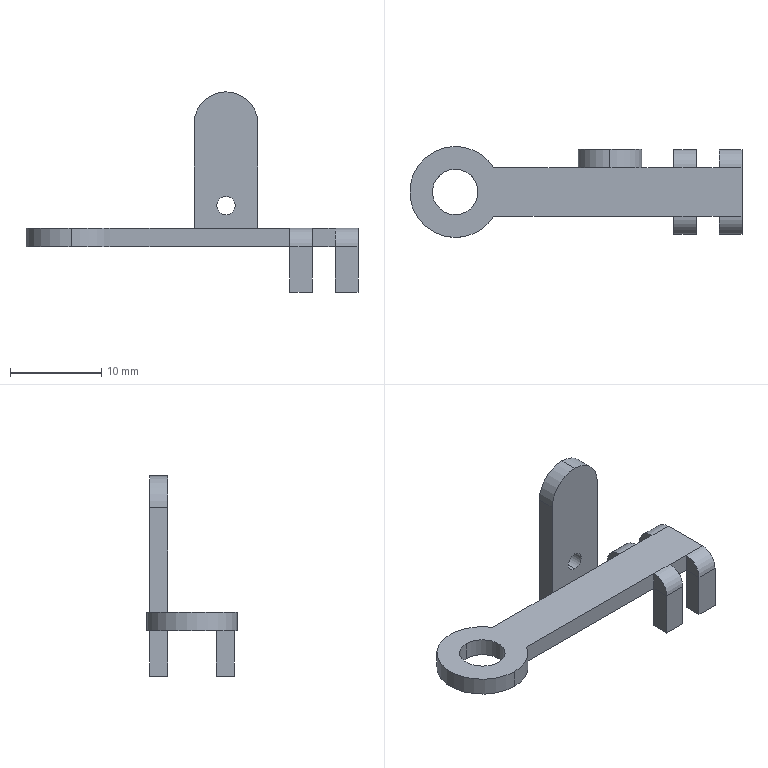Component | SolidWorks | BSH3-02-00ARubberBlankingAssembly2-1_BSH3-02-08BendingPlate-1 | 1 solid | 53 faces | volume 754 mm3 | plane 40 | cylinder 13 | commonest cylinder face diameters 4 x4 10 x3 2 x2 7 x2 5 x2